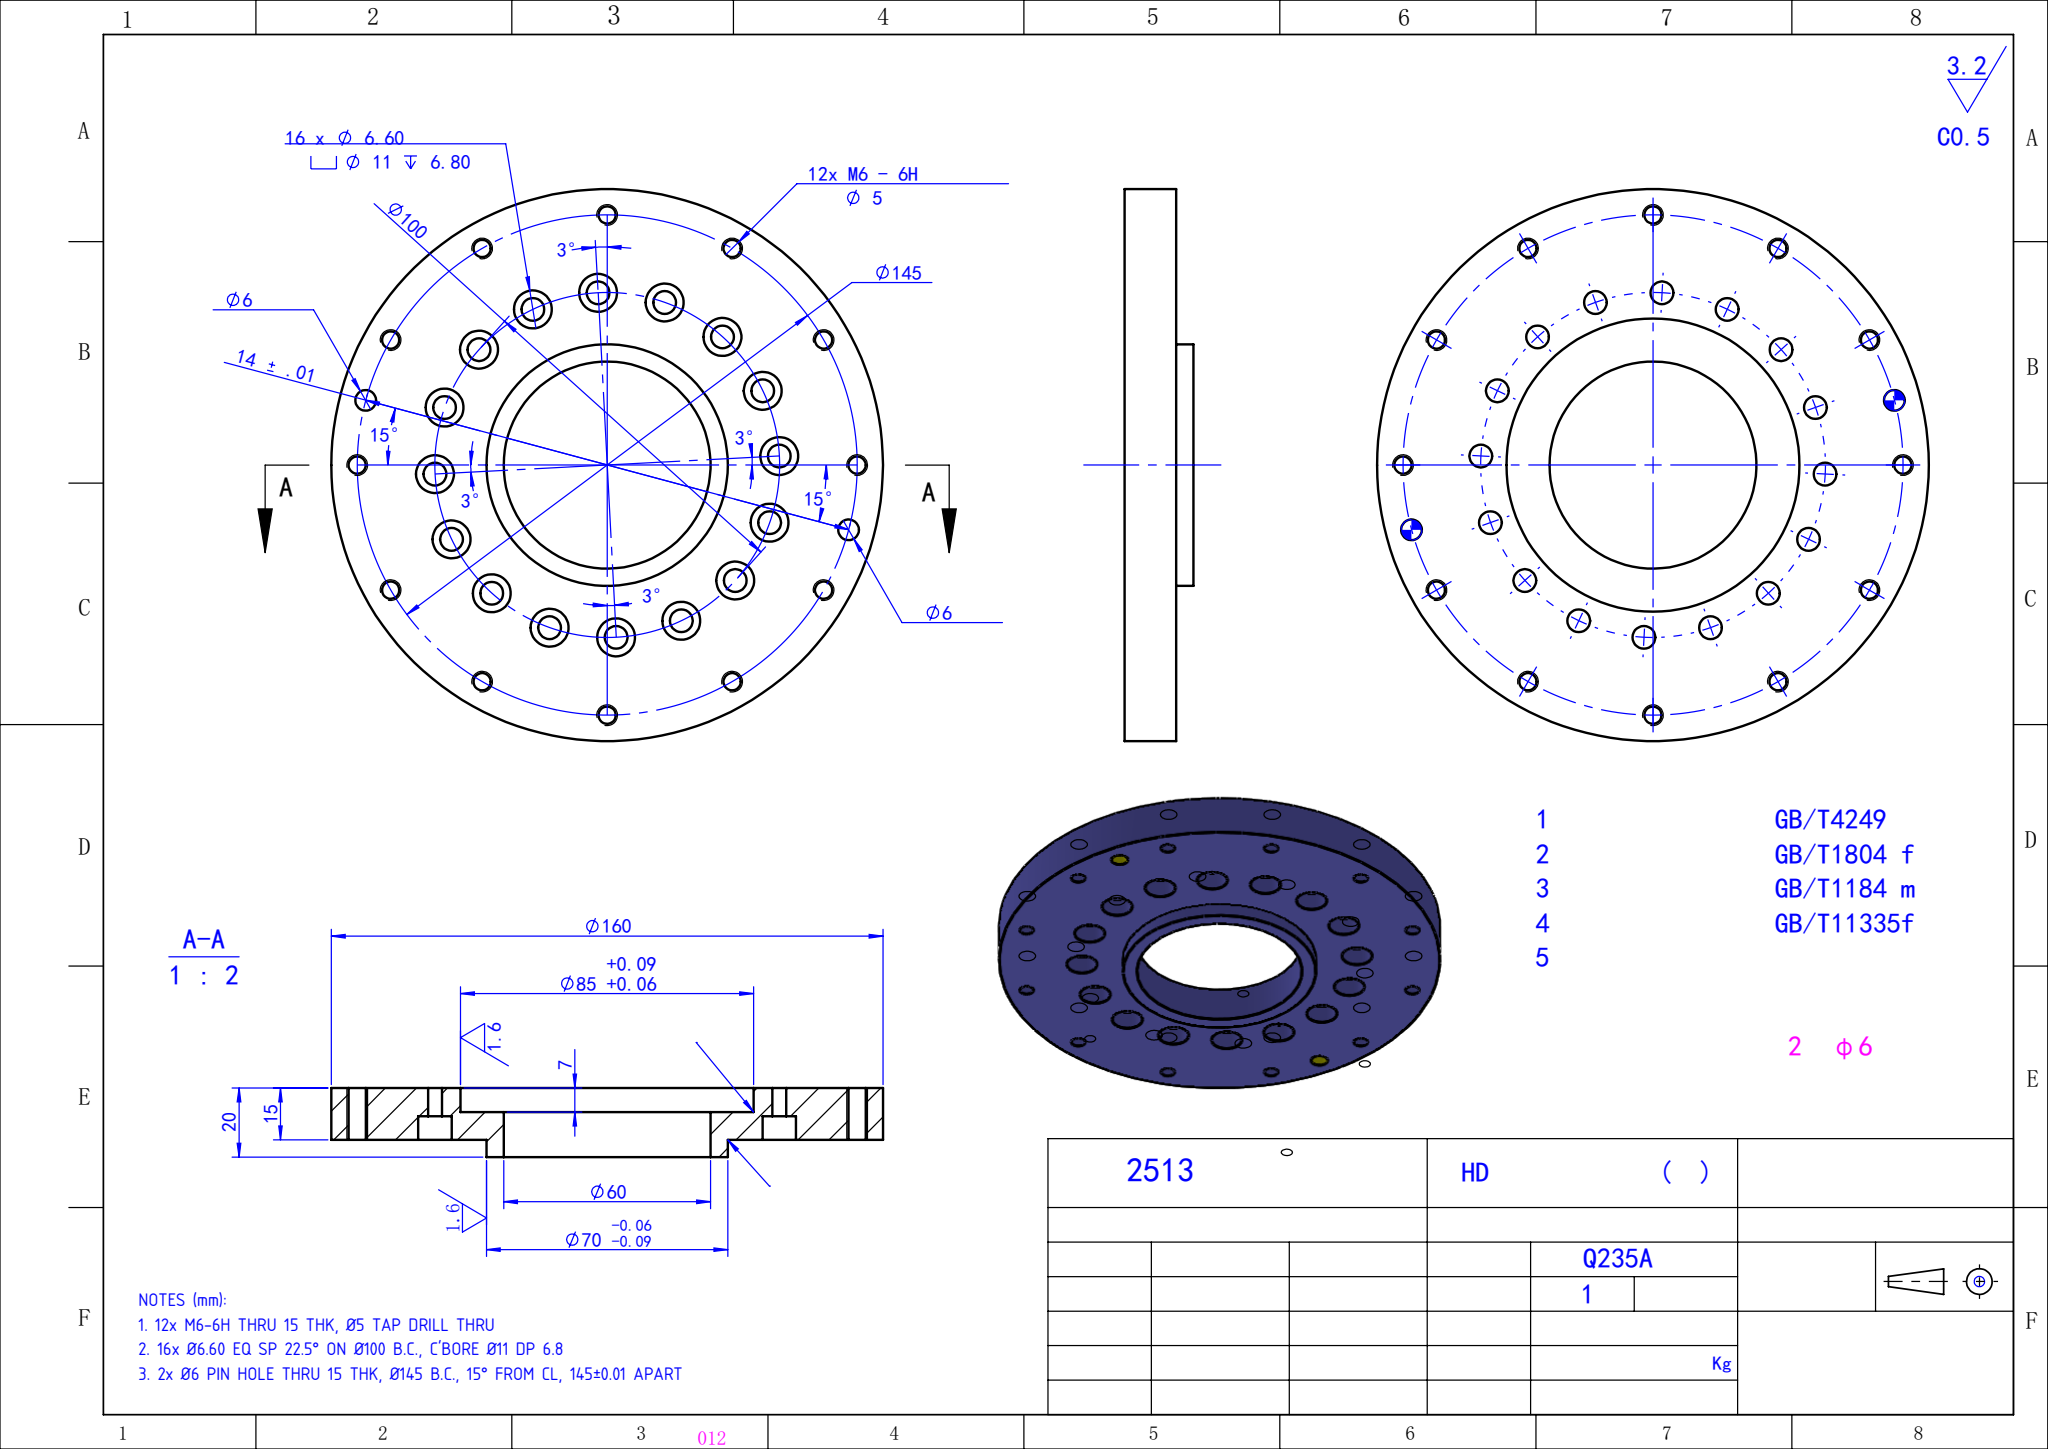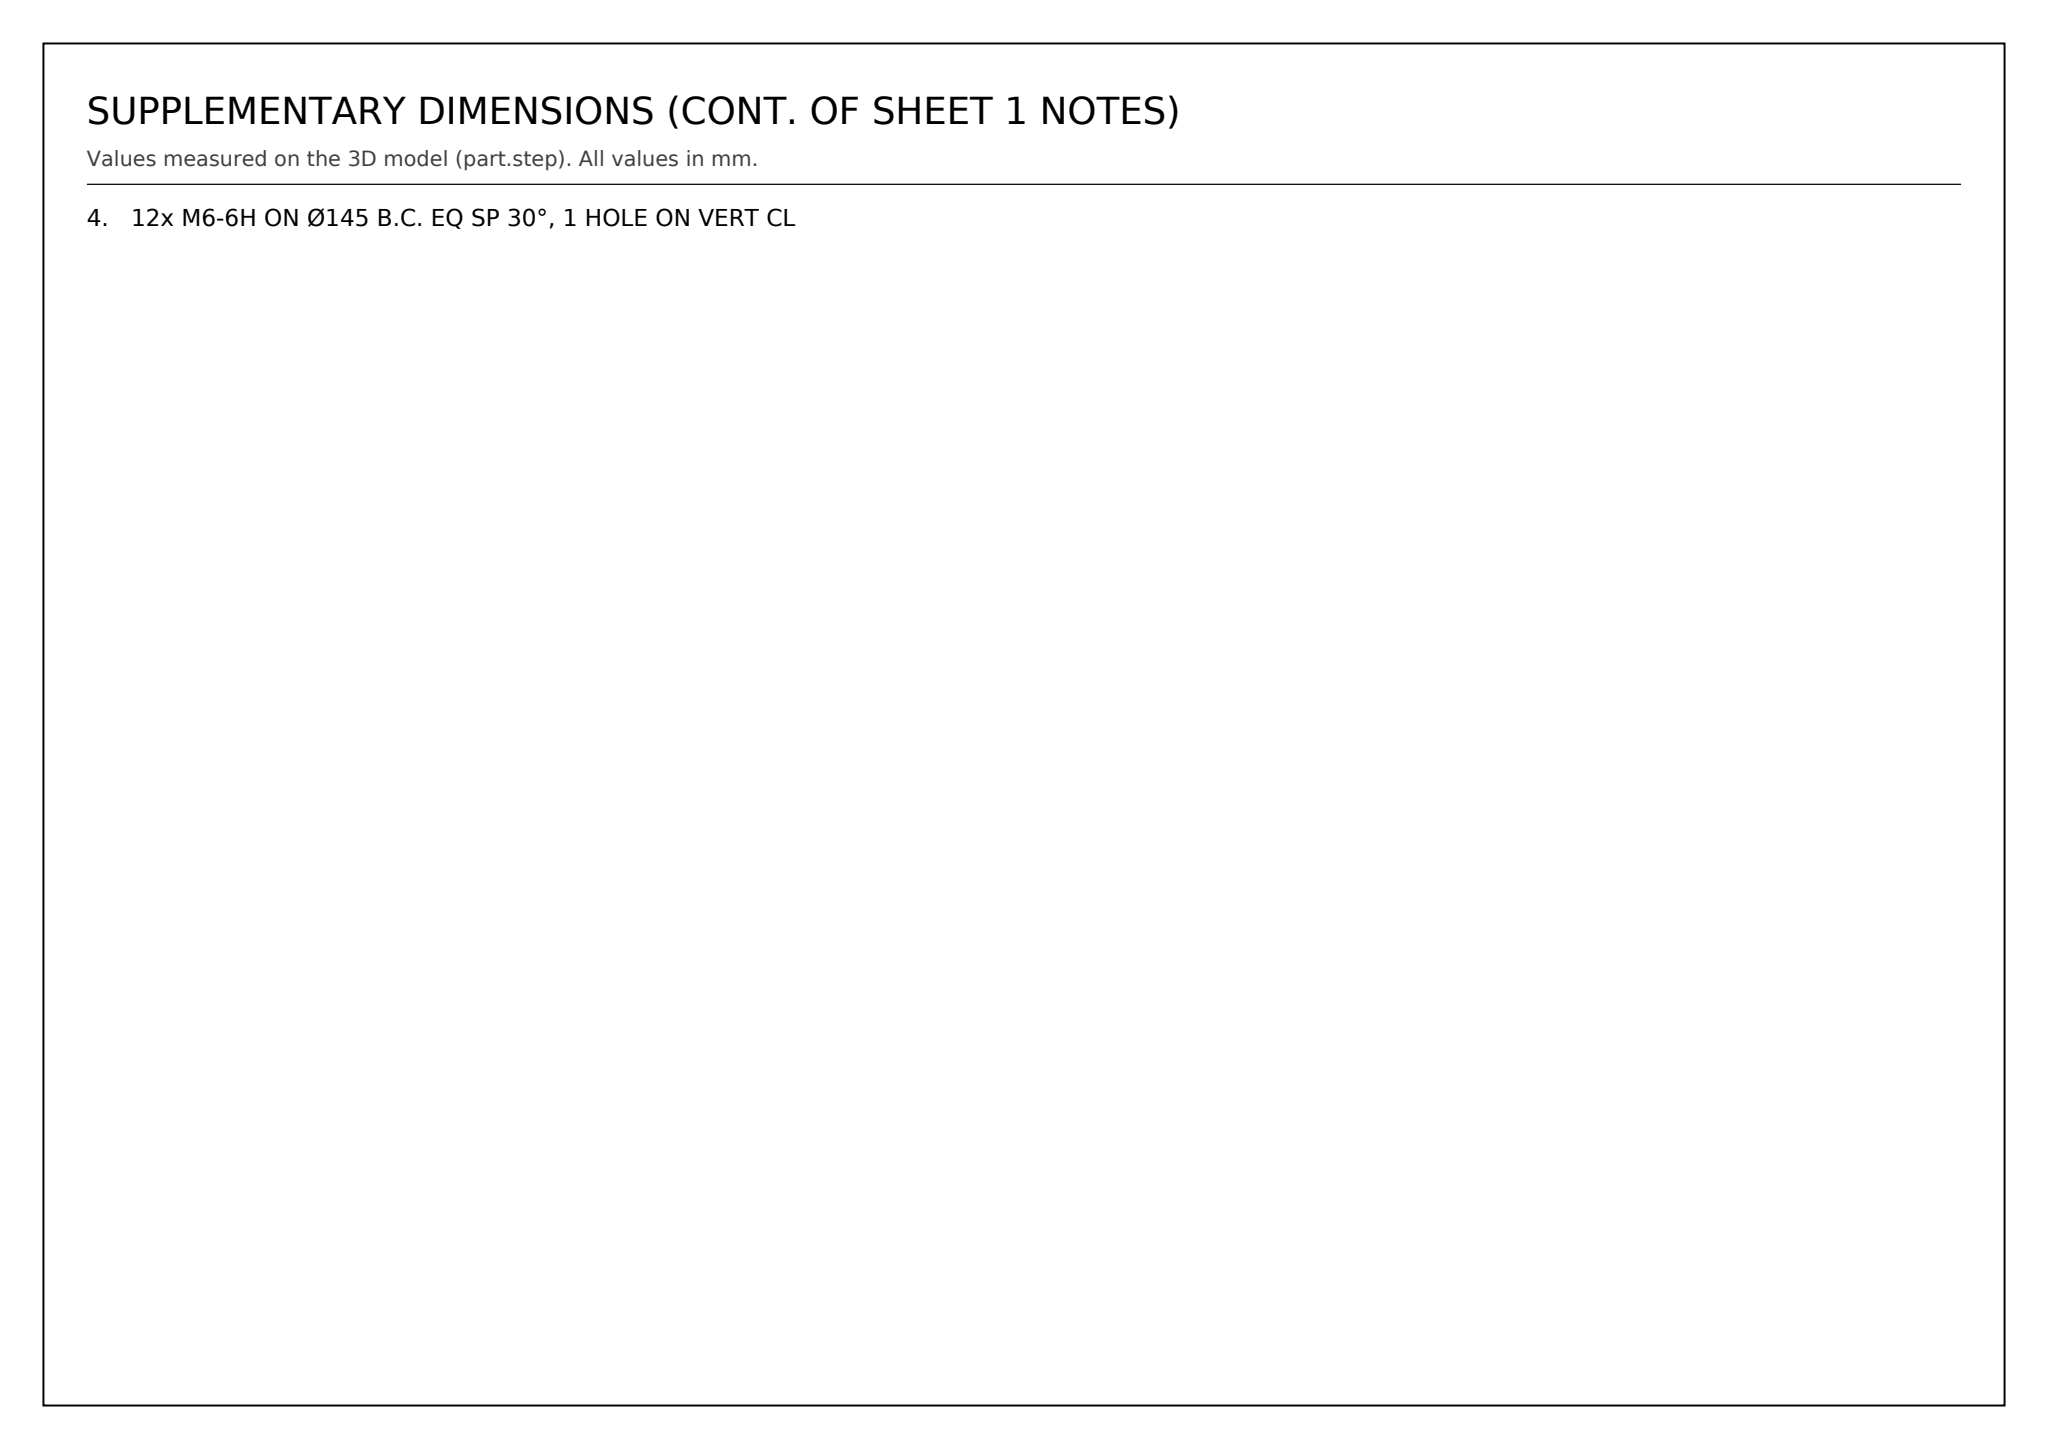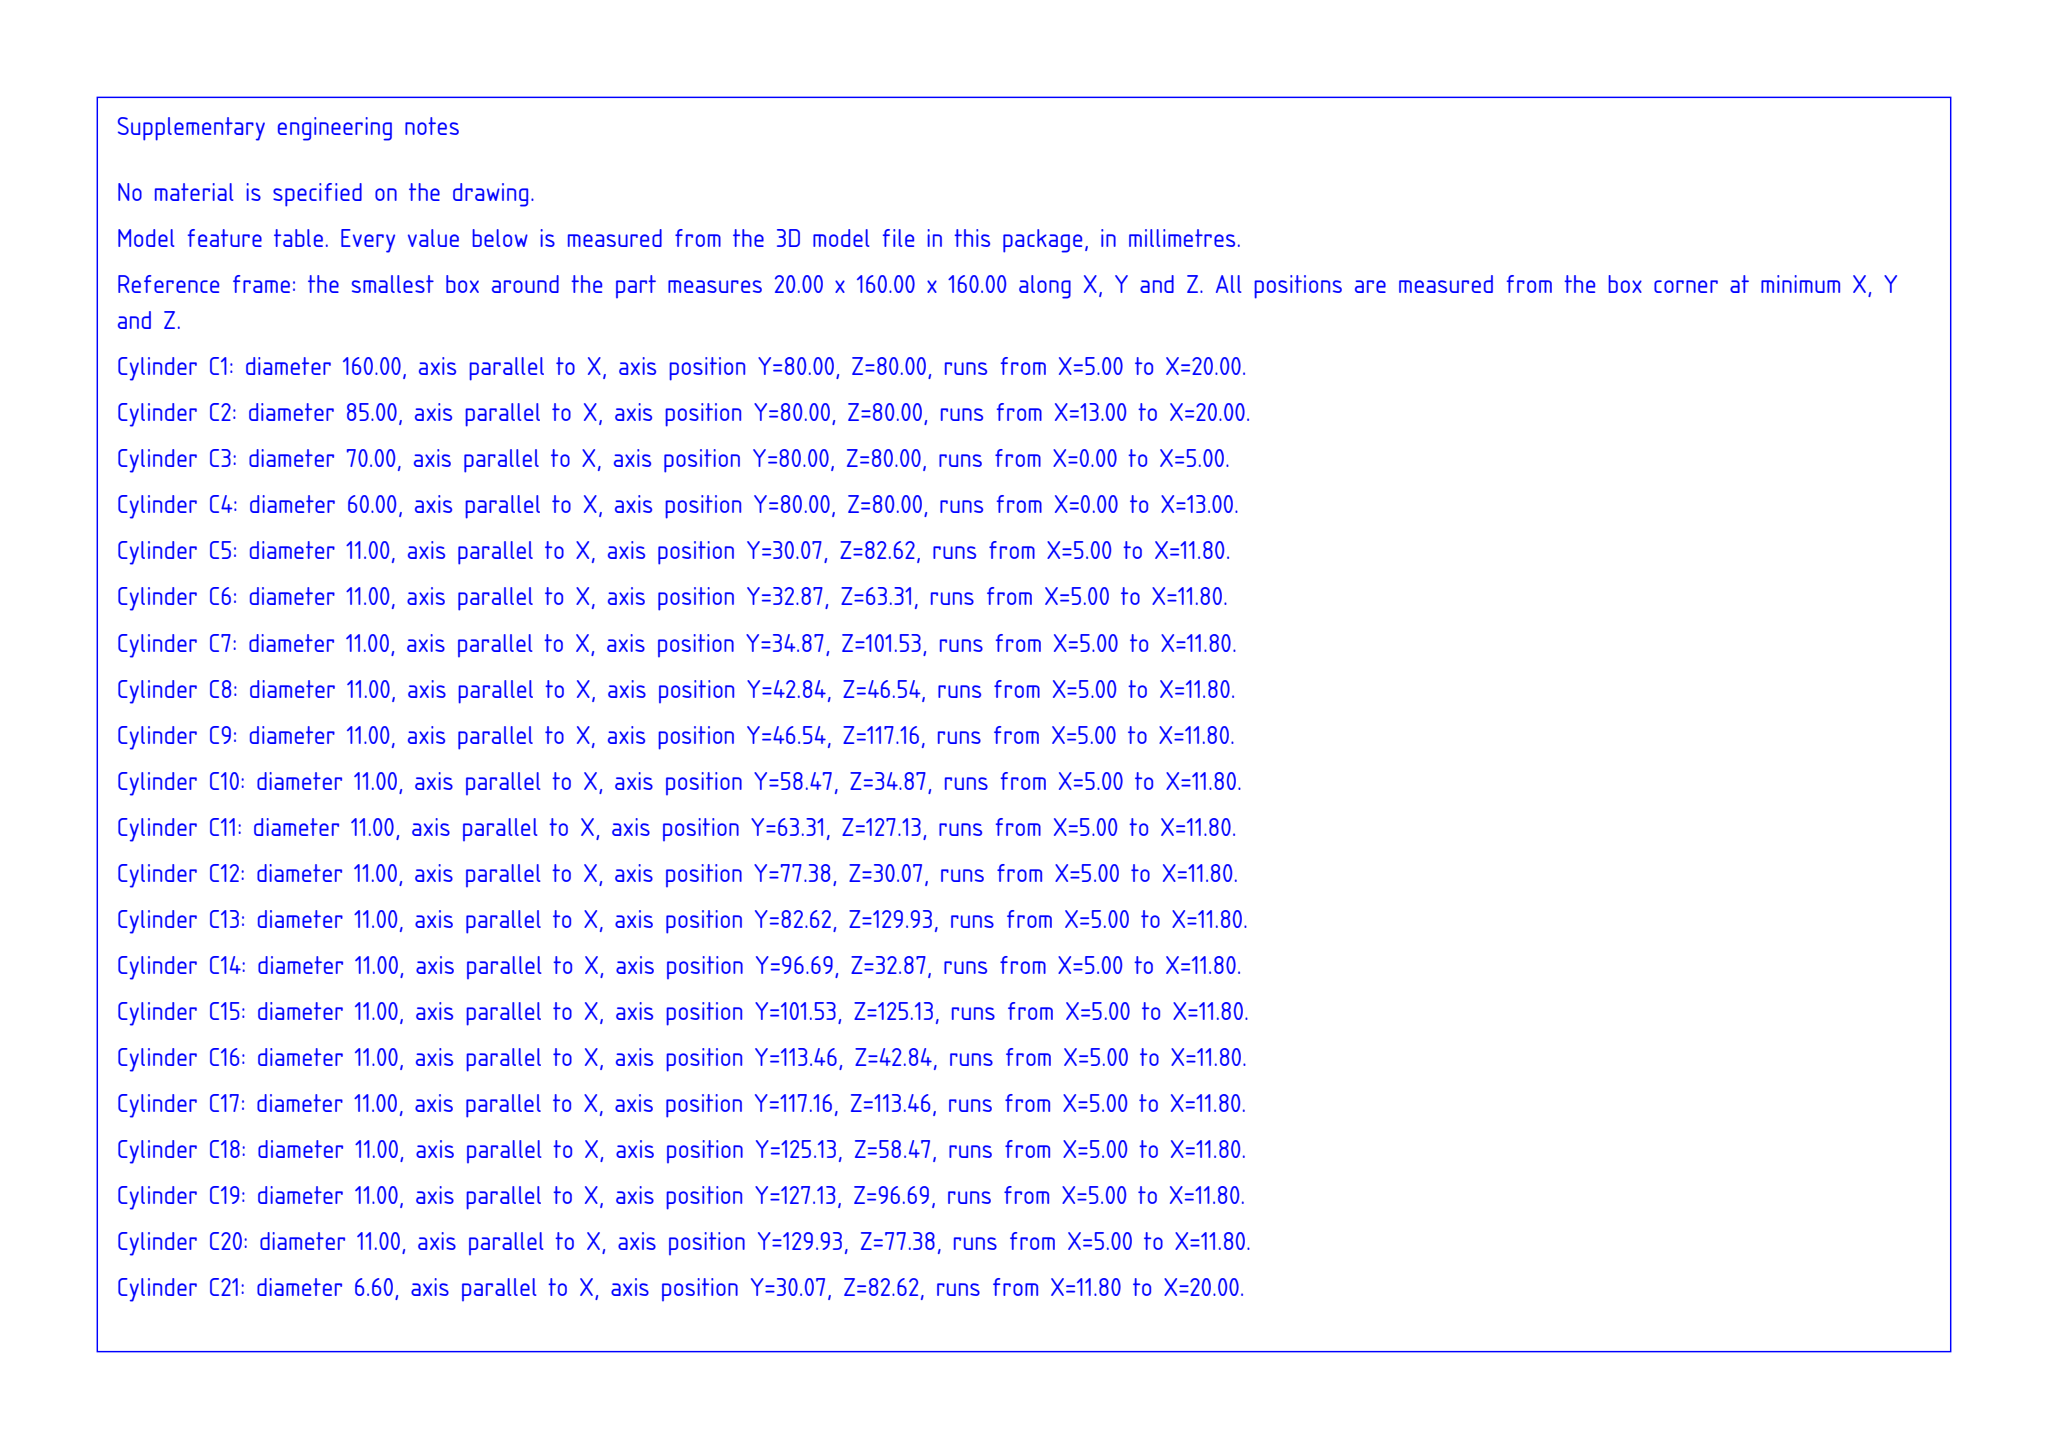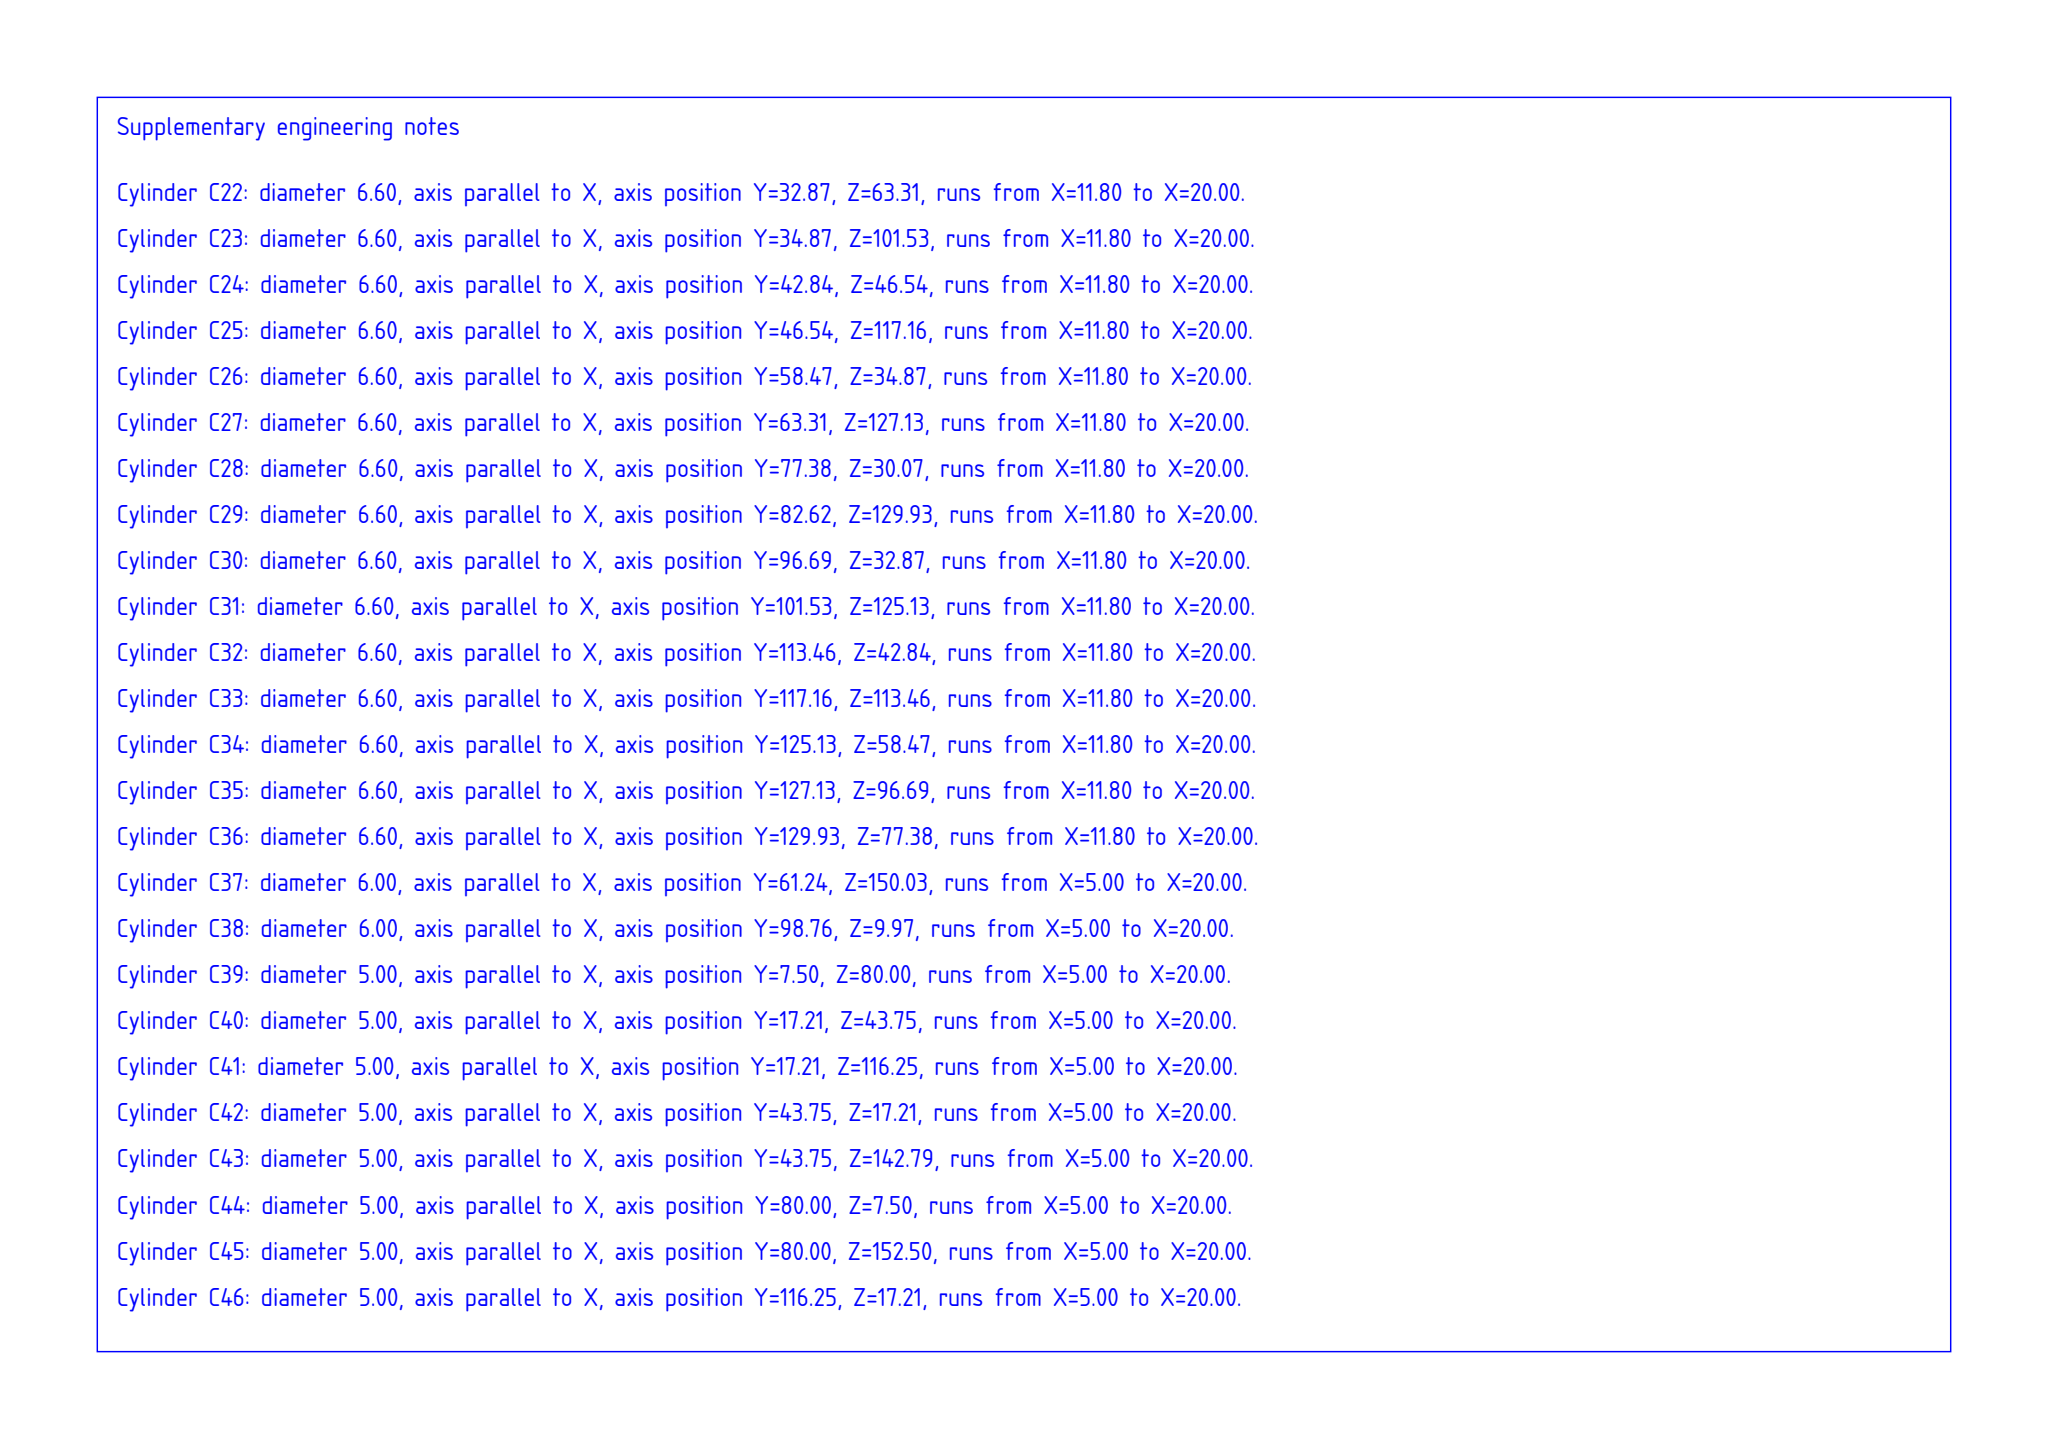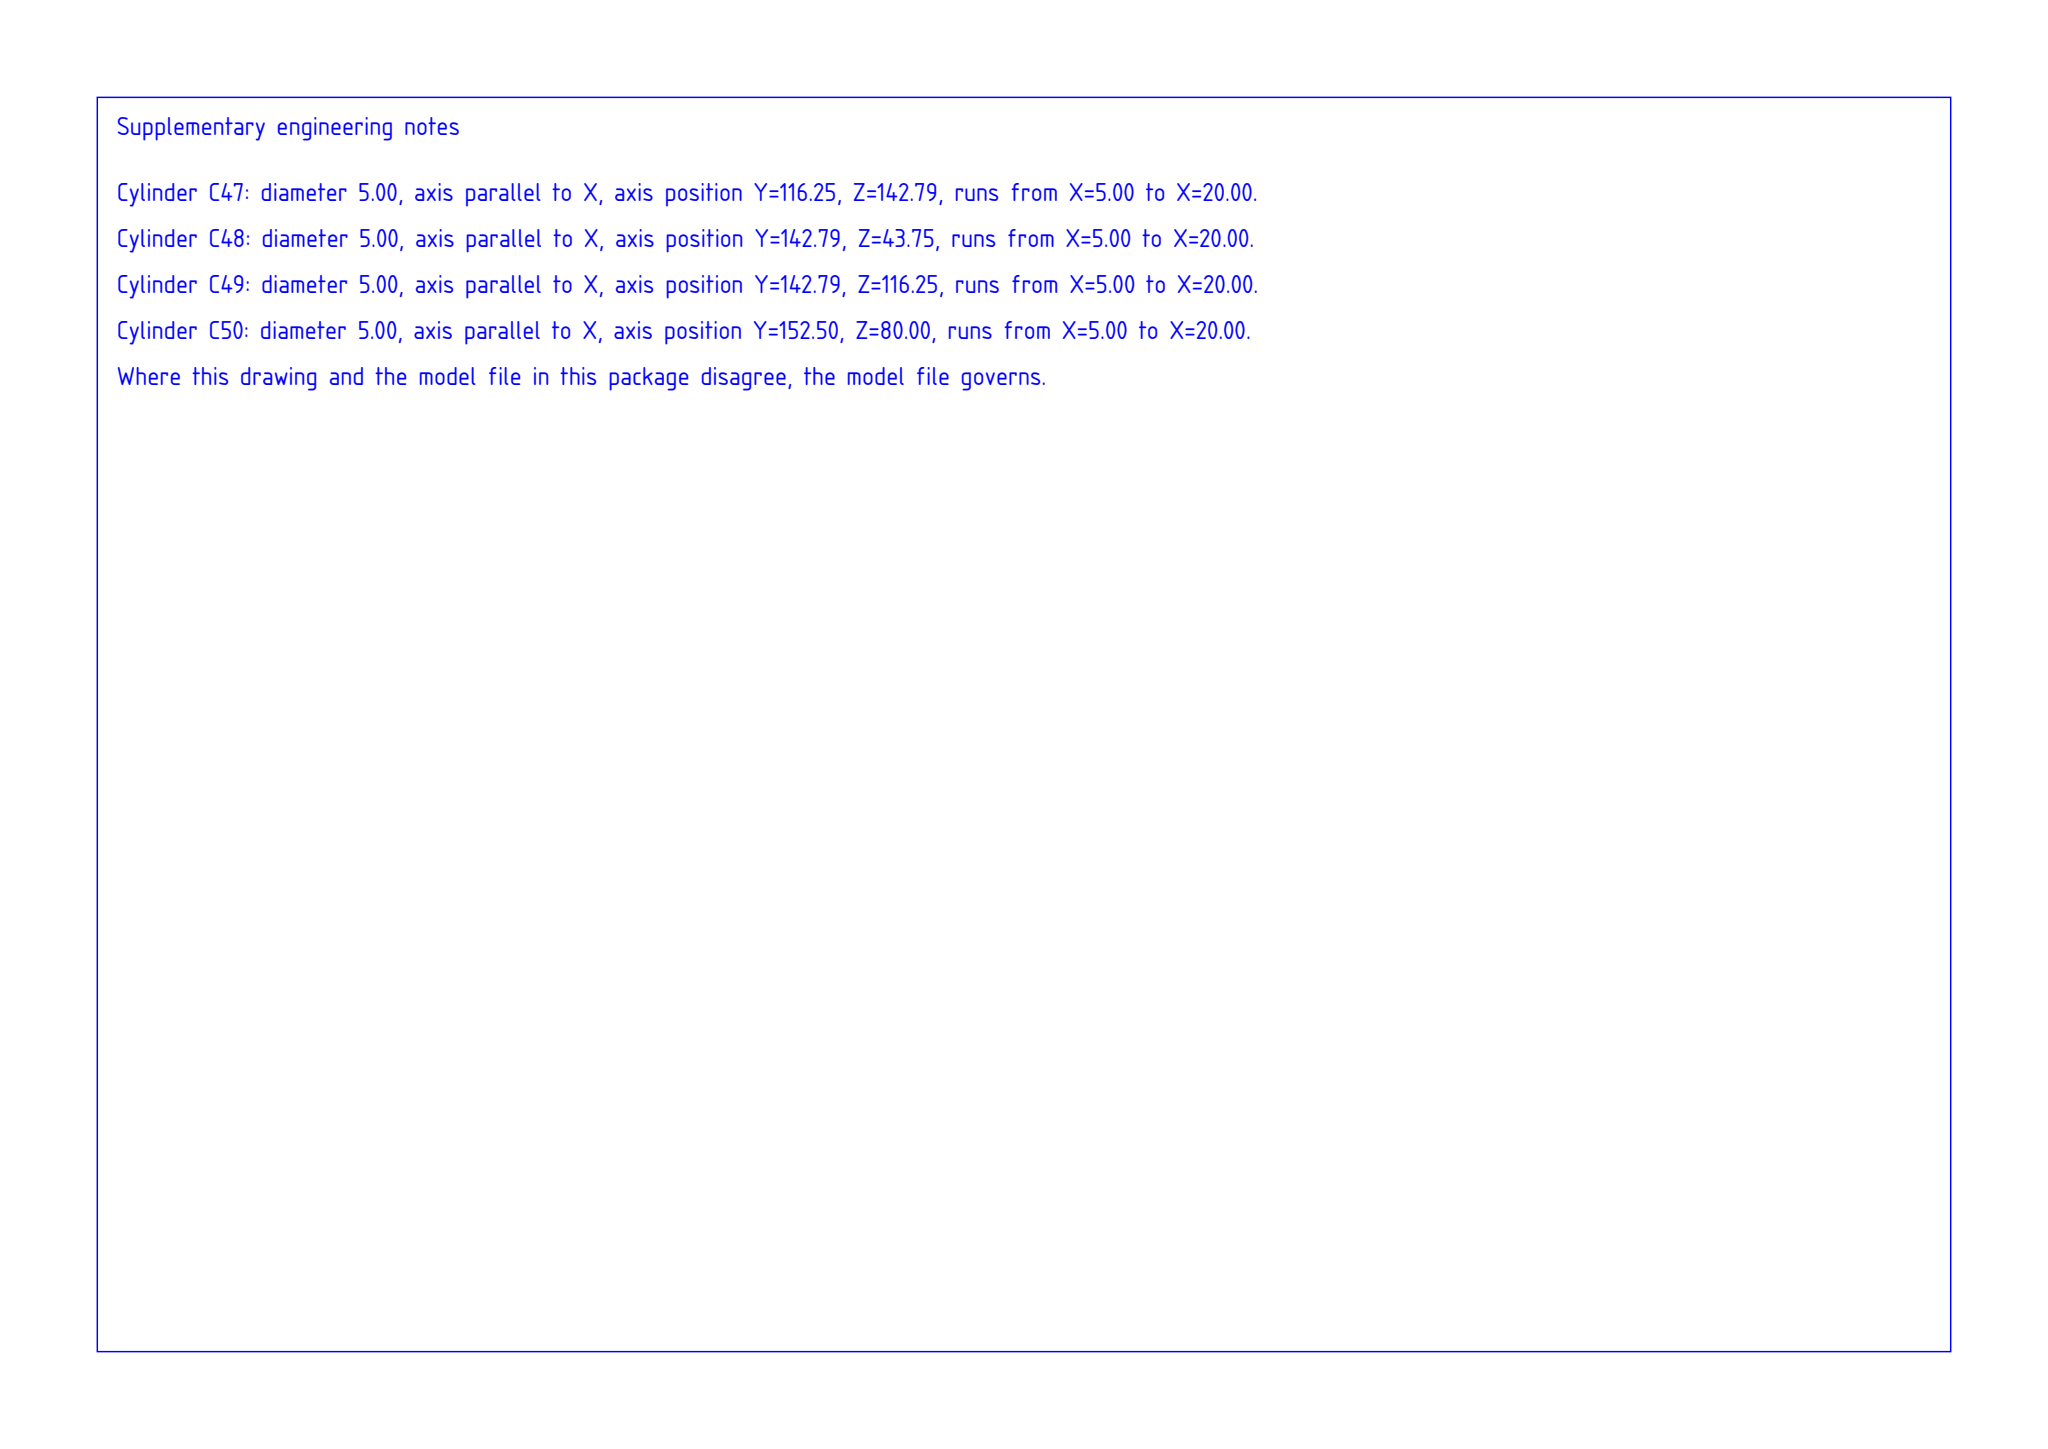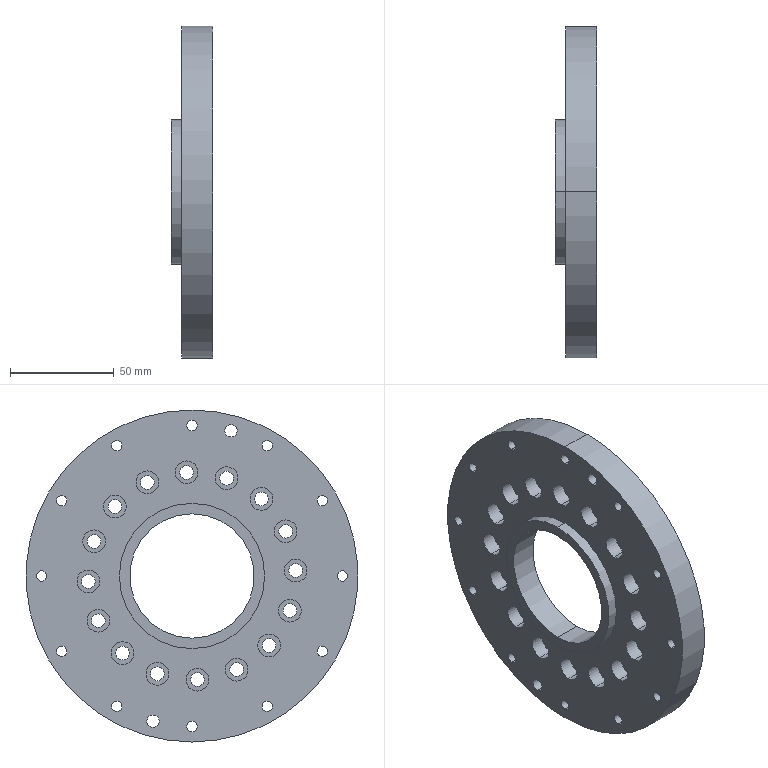Part | SolidWorks | mm | material Q235A | 1 solid | 120 faces | box 20 x 160 x 160 mm | volume 225146 mm3 | cylinder 100 | plane 20 | commonest cylinder face diameters 11 x32 6.6 x32 5 x24 6 x4 160 x2 60 x2 85 x2 70 x2
Drawing notes:
12x M6-6H THRU 15 THK, Ø5 TAP DRILL THRU | from the solid: Ø5 cylinders, axis x, length 15.0 = plate web thickness (x 0->15 region), 12 instances on Ø145 B.C.
16x Ø6.60 EQ SP 22.5° ON Ø100 B.C., C'BORE Ø11 DP 6.8 | from the solid: 16x Ø6.6 holes all at R50.0 from center (80,80); angular increments of 22.5°; Ø11 c'bores length 6.8
2x Ø6 PIN HOLE THRU 15 THK, Ø145 B.C., 15° FROM CL, 145±0.01 APART | from the solid: Ø6 holes at (61.24,150.03) & (98.76,9.97): R72.5 from center, 105° & 285° (15° off vert CL), length 15 thru; chord = 145
12x M6-6H ON Ø145 B.C. EQ SP 30°, 1 HOLE ON VERT CL | from the solid: Ø5 thru holes all at R72.5 from axis (80,80); e.g. (7.5,80),(17.21,43.75),(43.75,17.21),(80,7.5)...; adjacent angular step = 30°, one hole on Y centerline